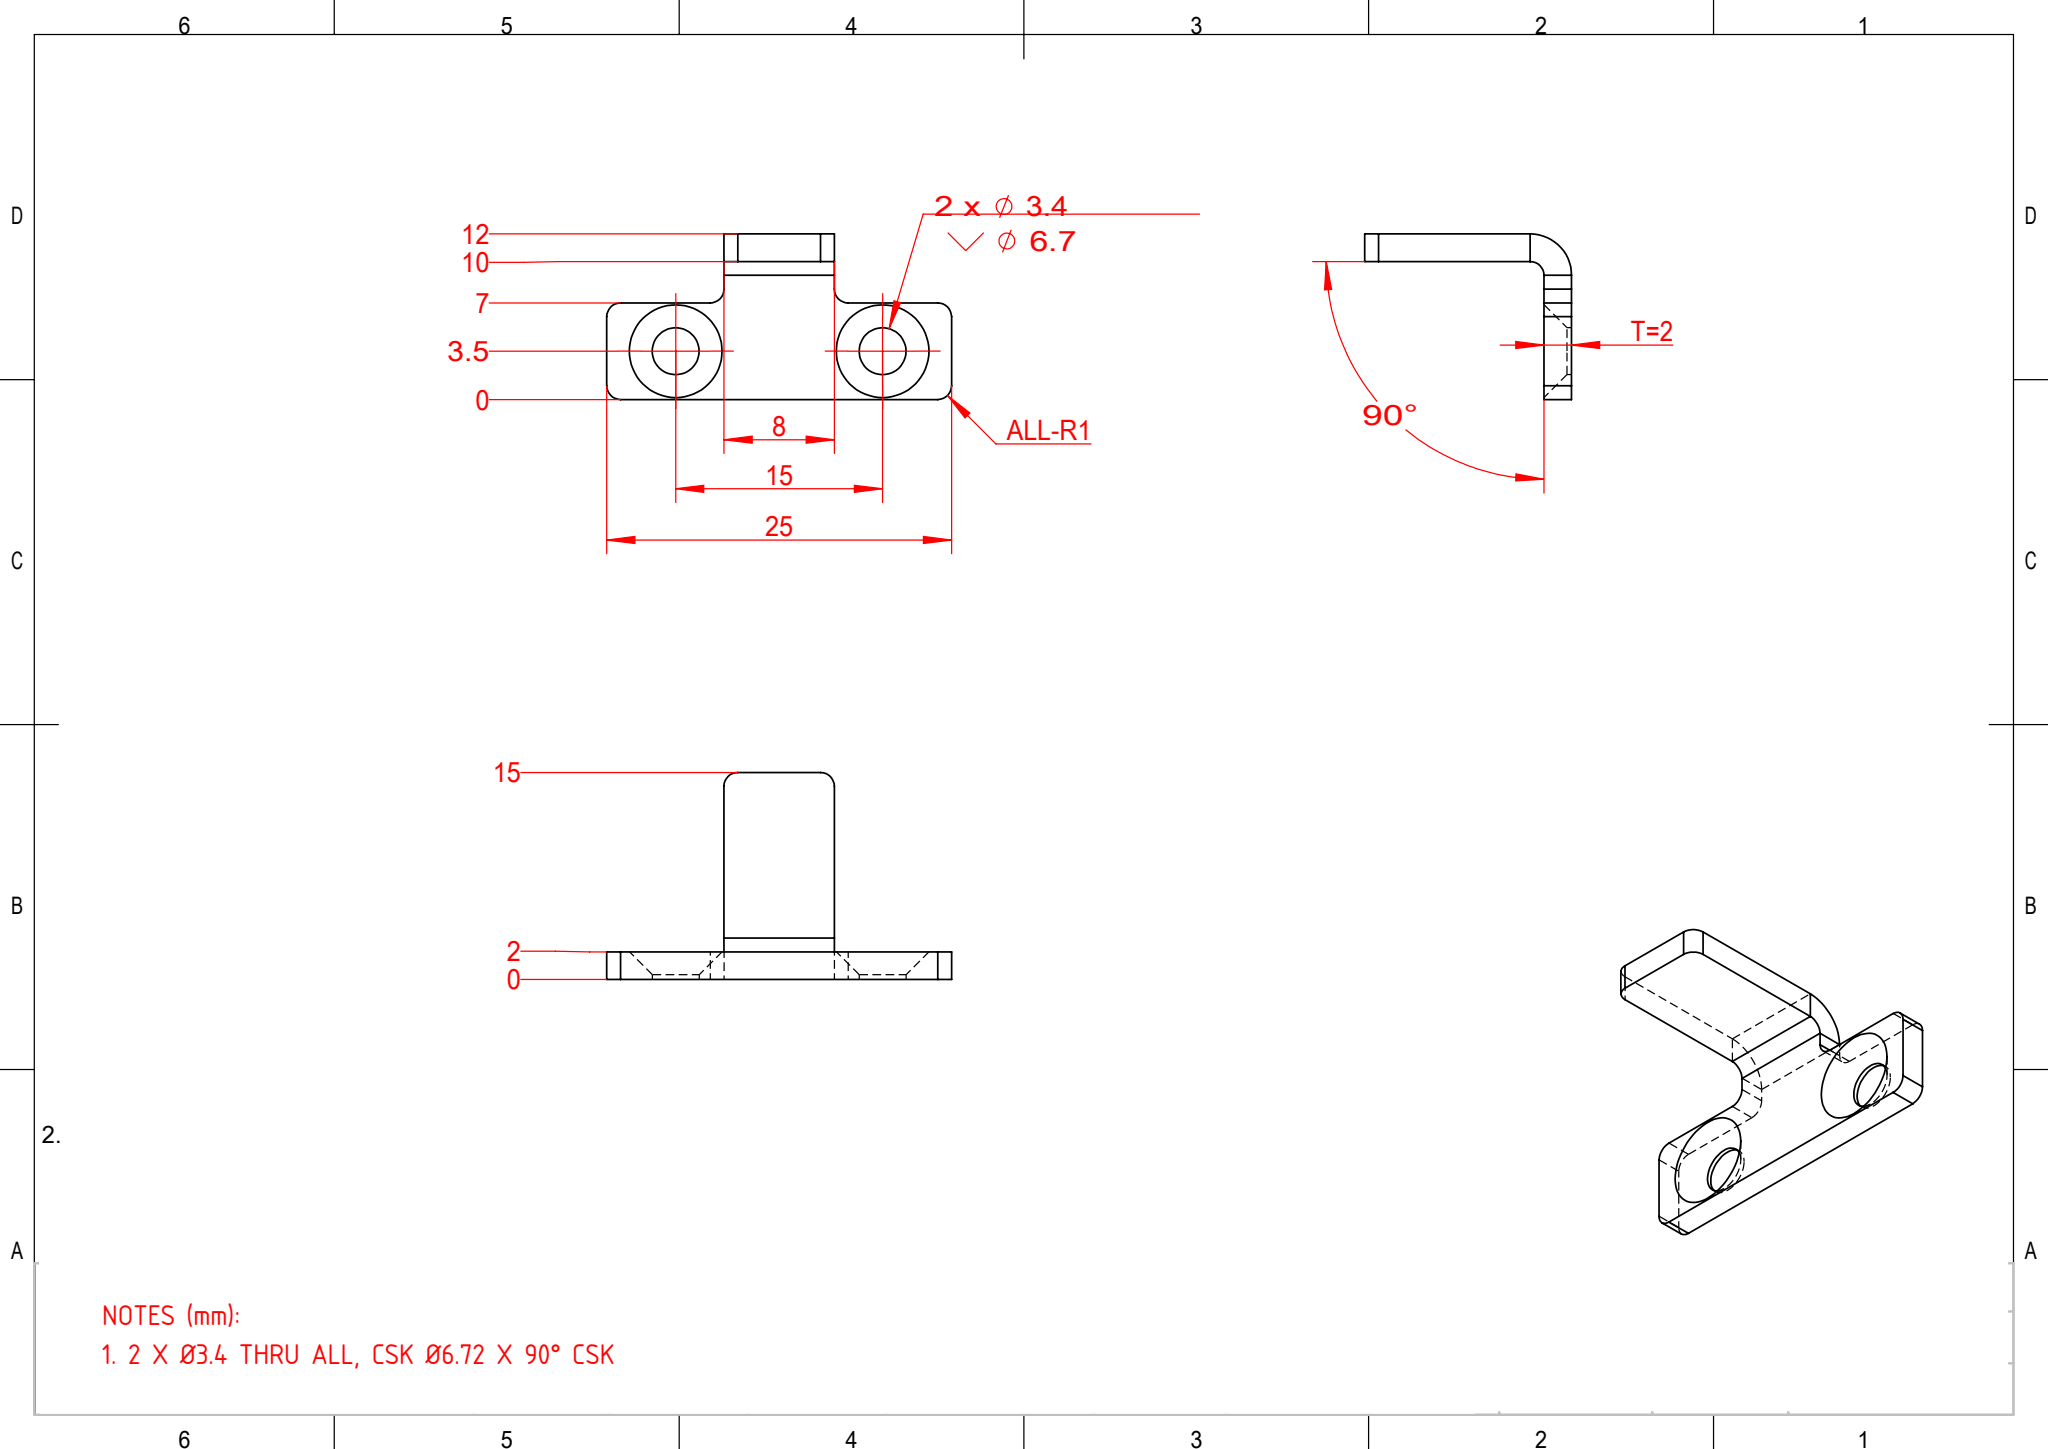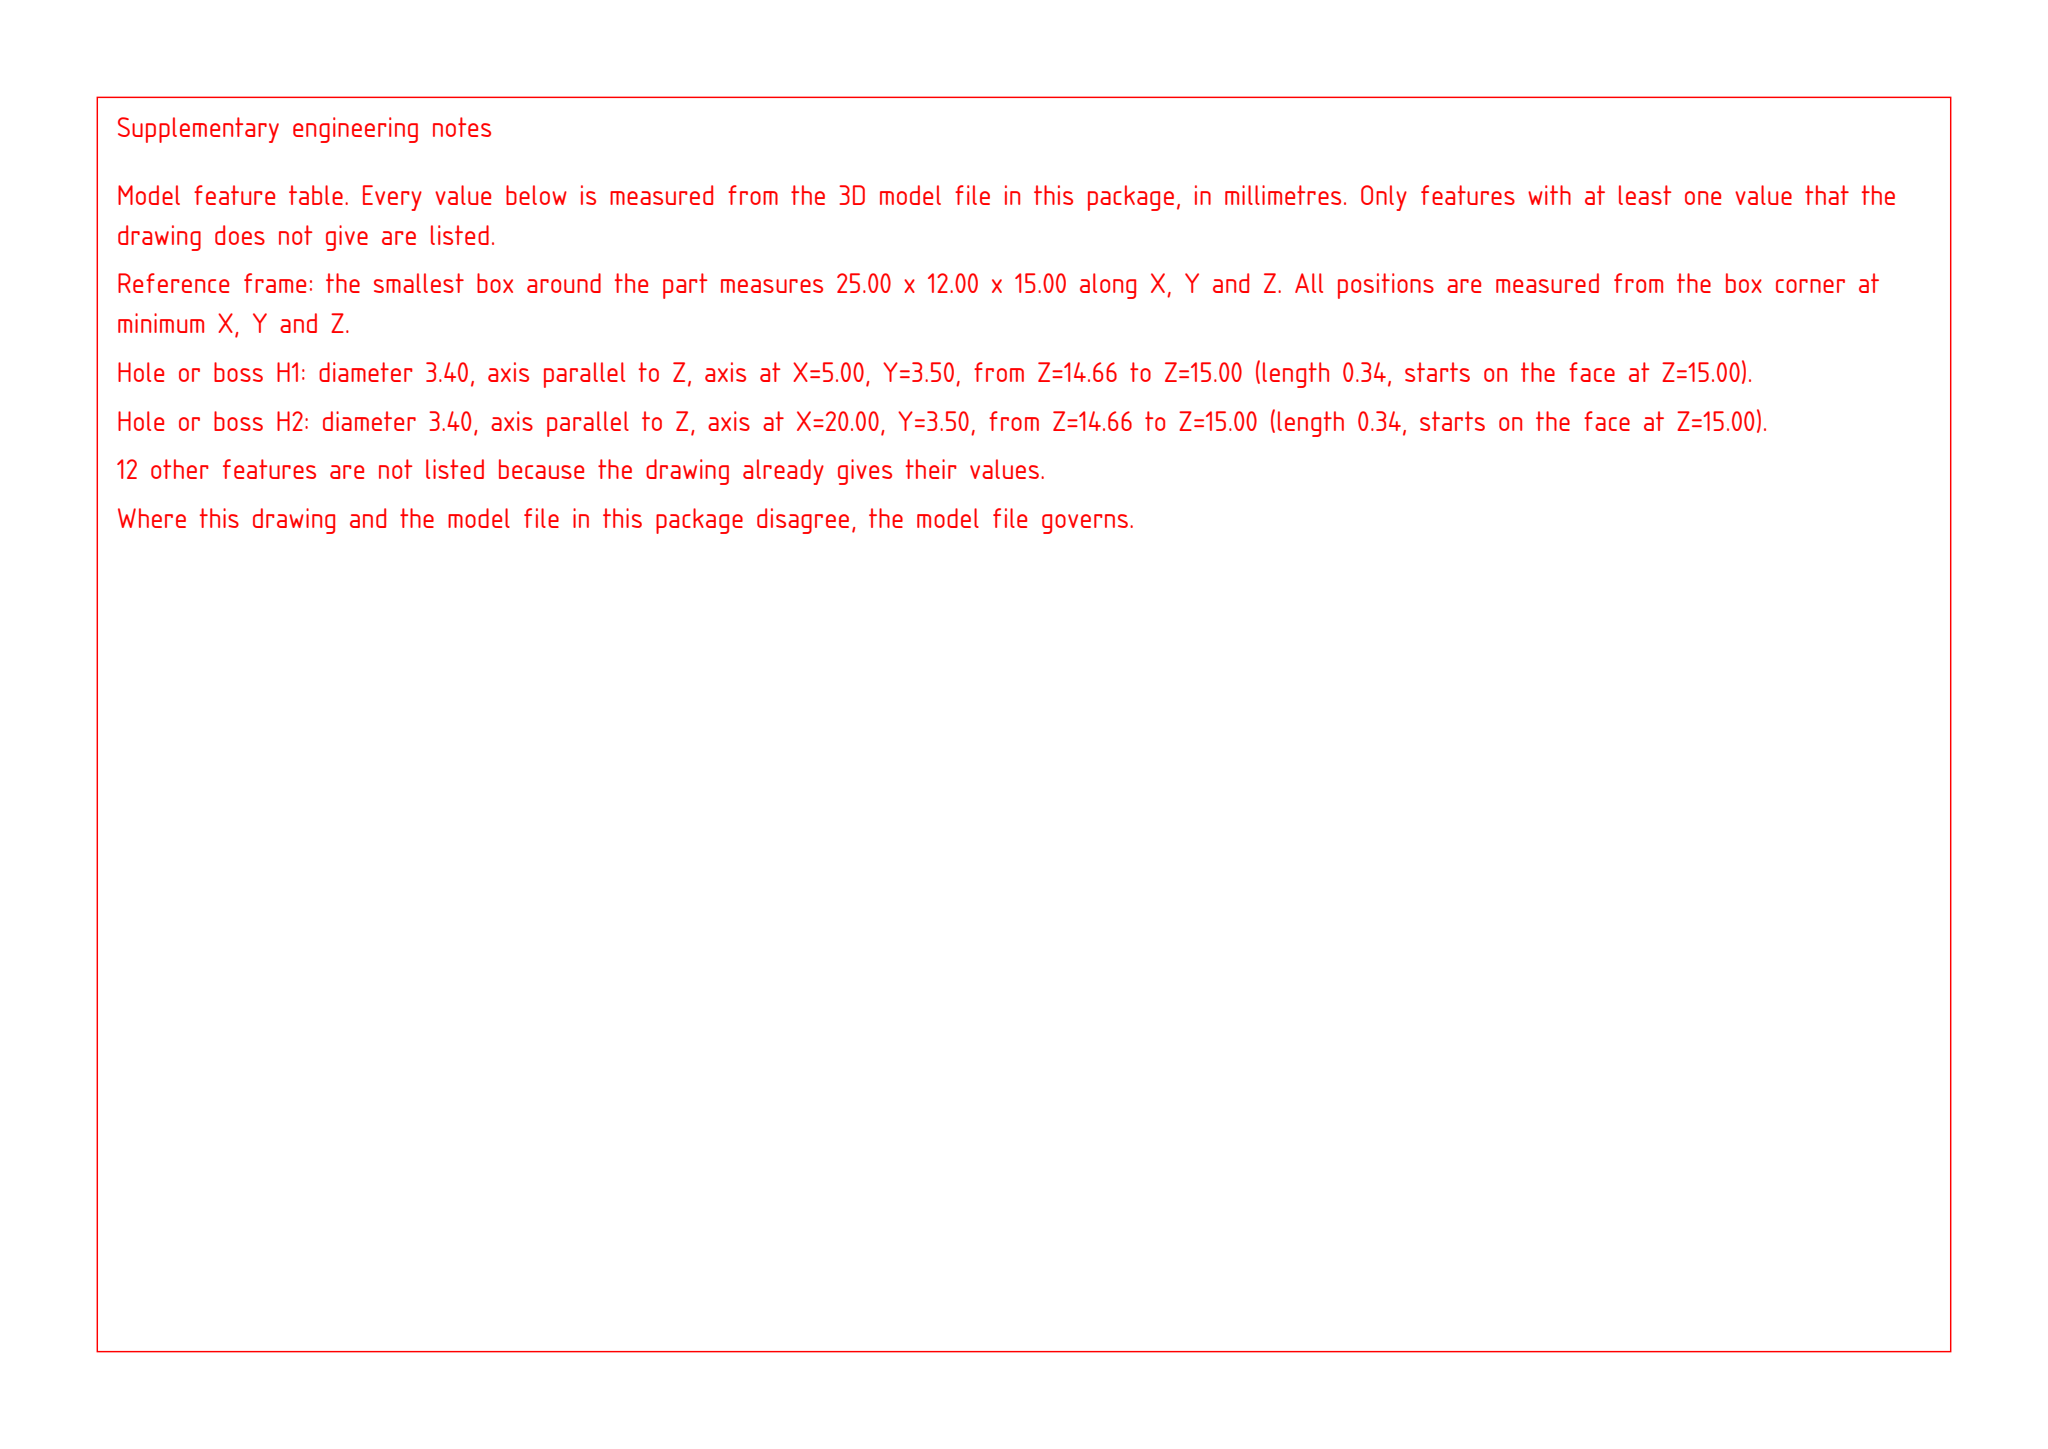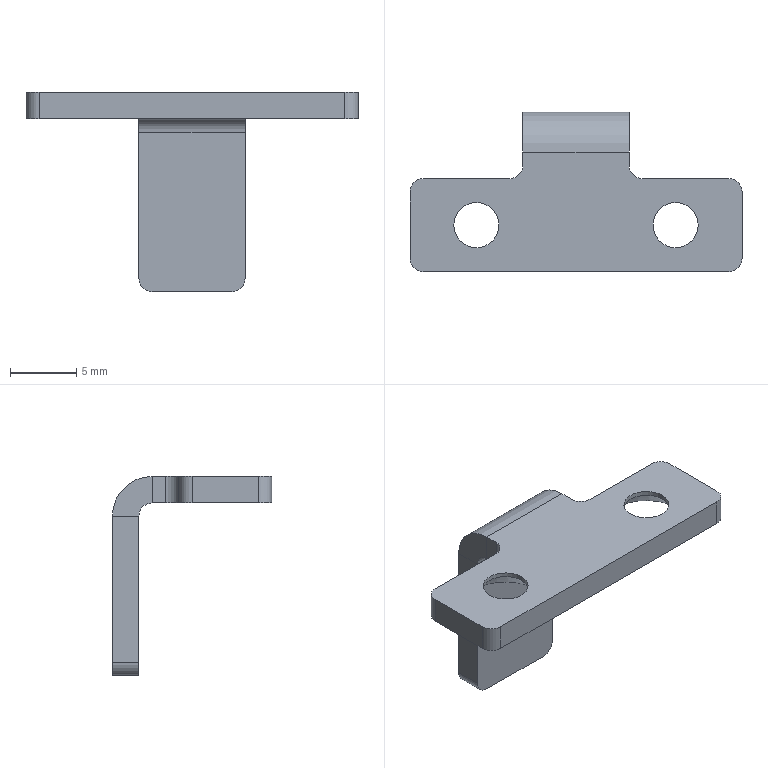Part | SolidWorks | mm | 1 solid | 34 faces | box 25 x 12 x 15 mm | volume 547 mm3 | plane 16 | cylinder 14 | cone 4 | commonest cylinder face diameters 2 x9 3.4 x4 6 x1
Drawing notes:
2 X Ø3.4 THRU ALL, CSK Ø6.72 X 90° CSK | from the solid: cones[included_angle,ref_dia]=[90.0,6.72] x4; Ø3.4 thru holes at (5.0,3.5) and (20.0,3.5)